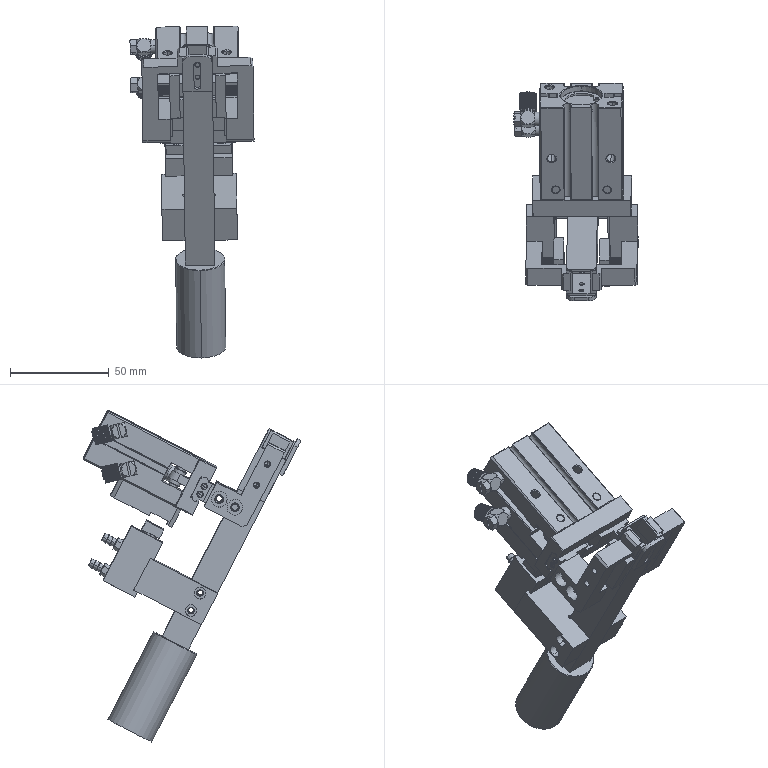Assembly | SolidWorks | mm | 18 component files | 21 solids | 1337 faces | box 62.86 x 110.43 x 168.21 mm | volume 158382 mm3 | plane 692 | cylinder 460 | cone 157 | spline 12 | sphere 12 | torus 4 | commonest cylinder face diameters 8.5 x72 2.5 x49 6 x38 3 x22 4.134 x20 5 x20 8 x20 4 x18
Bill of materials:
2018SOLIDWORKS1400000009 | 1 | 6061 Alloy | Rectangular block with a central rectangular slot that splits one end into two legs (a U/fork shape). It has a shallow step or lip along the top edges, small round relief grooves at the inner corners of the slot, and cross holes through the legs.
2018SOLIDWORKS1400000010 | 1 | 45 Steel | Long, narrow flat bar or channel that comes out of a short solid cylinder at one end. The far end splits into two thin prongs with small holes, and there is a pair of small holes partway along the bar.
2018SOLIDWORKS1400000011 | 1 | Black POM | Flat rectangular plate with two rounded corners on one end and one long obround slot through it.
2018SOLIDWORKS1400000012 | 1 | 45 Steel | L-shaped stepped bracket with an extra notched tab at the tip of one arm. Several through holes run through the plate-like face, some with counterbore-like rims.
2018SOLIDWORKS1400000013 | 1 | 45 Steel | L-shaped stepped bracket with a notched tab at one arm end. It has two larger counterbored-looking holes at the corner end and two smaller holes along the long arm.
2018SOLIDWORKS1400000014 | 2 | White High Temperature Silicone | Plain rectangular block or thick plate with a shallow narrow rectangular step or groove near one edge.
2018SOLIDWORKS1400000015 | 2 | 45 Steel | Plain rectangular block or thick plate with no visible holes or other features.
2018SOLIDWORKS1400000016 | 1 | 6061 Alloy | Rectangular plate with chamfered corners. It has two plain through holes, two counterbored holes, and a stepped notch along one edge.
PurchasedPart;Three-axisCylinderTCM10x5S | 1 |  | Rectangular block with two parallel vertical slots that have semicircular ends. It also has a lateral groove, a row of holes and counterbores on one face, and side holes. A thin plate on a short neck stands off one end.
PurchasedPart_5mmSmallSpring | 2 |  | Helical coil of round wire with many evenly spaced turns. A solid cylinder sits inside part of its length.
PurchasedPart_MiniConnector03-_4 | 2 |  | Axially symmetric tubular fitting-like part. It has a hex flange, a short plain spigot on one side and a tapered, ringed (barb-like) stem on the other, with a through bore.
PurchasedPart_MS-5HLH-6StainlessSteelConnector | 2 |  | Compact body with a rounded or spherical central section. A hex section with a slot sits on one side and a stepped cylindrical nozzle with a bore on the opposite side. A large knurled or fluted cylindrical knob comes out at a right angle.
Y0365088900012 | 1 |  | Rectangular prismatic body with a wider transverse plate across one end. Two parallel rectangular jaw-like fingers stick out of that end. The overall shape looks like a two-finger parallel gripper unit.
Mates:
1. distance | 2018SOLIDWORKS1400000015-1 face at (82.559, -98.378, 177.003) dir (-0.9999, 0, -0.01383) | 2018SOLIDWORKS1400000012-1 face at (76.322, -113.007, 194.123) dir (0.9999, 0, 0.01383)
2. concentric | 2018SOLIDWORKS1400000012-1 face at (70.561, -98.378, 176.837) dir (0.9999, 0, 0.01383) r 3 | 2018SOLIDWORKS1400000015-1 face at (85.559, -98.378, 177.045) dir (-0.9999, 0, -0.01383) r 2.5
3. parallel | 2018SOLIDWORKS1400000012-1 face at (68.765, -96.483, 162.032) dir (0.00635, -0.8884, -0.459) | 2018SOLIDWORKS1400000015-1 face at (82.755, -99.533, 162.901) dir (0.00635, -0.8884, -0.459)
4. coincident | 2018SOLIDWORKS1400000012-1 face at (75.885, -87.155, 153.442) dir (0.9999, 0, 0.01383) | Y0365088900012-1 face at (75.284, -13.933, 196.896) dir (-0.9999, 0, -0.01383)
5. concentric | 2018SOLIDWORKS1400000012-1 face at (68.79, -84.741, 160.22) dir (-0.9999, 0, -0.01383) r 2.25 | Y0365088900012-1 face at (79.794, -84.741, 160.372) dir (0.9999, 0, 0.01383) r 1.621
6. concentric | 2018SOLIDWORKS1400000012-1 face at (68.733, -76.745, 164.351) dir (-0.9999, 0, -0.01383) r 2.25 | Y0365088900012-1 face at (79.737, -76.745, 164.503) dir (0.9999, 0, 0.01383) r 1.621
7. coincident | Y0365088900012-1 face at (117.579, -13.933, 197.481) dir (0.9999, 0, 0.01383) | 2018SOLIDWORKS1400000013-1 face at (118.072, -82.786, 161.912) dir (-0.9999, 0, -0.01383)
8. concentric | Y0365088900012-1 face at (114.024, -76.745, 164.977) dir (0.9999, 0, 0.01383) r 1.621 | 2018SOLIDWORKS1400000013-1 face at (125.028, -76.745, 165.129) dir (0.9999, 0, 0.01383) r 2.25
9. concentric | Y0365088900012-1 face at (114.081, -84.741, 160.846) dir (0.9999, 0, 0.01383) r 1.621 | 2018SOLIDWORKS1400000013-1 face at (125.085, -84.741, 160.999) dir (0.9999, 0, 0.01383) r 2.25
10. distance | 2018SOLIDWORKS1400000015-2 face at (110.859, -98.645, 177.257) dir (0.9999, 0, 0.01383) | 2018SOLIDWORKS1400000013-1 face at (116.618, -113.007, 194.681) dir (-0.9999, 0, -0.01383)
11. concentric | 2018SOLIDWORKS1400000013-1 face at (122.857, -98.645, 177.423) dir (-0.9999, 0, -0.01383) r 3 | 2018SOLIDWORKS1400000015-2 face at (107.859, -98.645, 177.216) dir (0.9999, 0, 0.01383) r 2.5
12. parallel | 2018SOLIDWORKS1400000015-1 face at (82.755, -99.533, 162.901) dir (0.00635, -0.8884, -0.459) | 2018SOLIDWORKS1400000015-2 face at (111.054, -99.8, 163.155) dir (0.00635, -0.8884, -0.459)
13. concentric | 2018SOLIDWORKS1400000013-1 face at (122.857, -98.645, 177.423) dir (-0.9999, 0, -0.01383) r 3 | PurchasedPart_5mmSmallSpring-2 face at (117.858, -98.645, 177.354) dir (0.9999, 0, 0.01383) r 1.5
14. coincident | 2018SOLIDWORKS1400000013-1 face at (122.857, -98.645, 177.423) dir (-0.9999, 0, -0.01383) | PurchasedPart_5mmSmallSpring-2 face at (122.857, -98.645, 177.423) dir (0.9999, 0, 0.01383)
15. concentric | 2018SOLIDWORKS1400000012-1 face at (70.561, -98.378, 176.837) dir (0.9999, 0, 0.01383) r 3 | PurchasedPart_5mmSmallSpring-1 face at (75.56, -98.378, 176.907) dir (-0.9999, 0, -0.01383) r 1.5
16. coincident | 2018SOLIDWORKS1400000012-1 face at (70.561, -98.378, 176.837) dir (0.9999, 0, 0.01383) | PurchasedPart_5mmSmallSpring-1 face at (70.561, -98.378, 176.837) dir (-0.9999, 0, -0.01383)
17. coincident | 2018SOLIDWORKS1400000012-1 face at (88.833, -112.548, 193.408) dir (0.01229, 0.459, -0.8883) | 2018SOLIDWORKS1400000014-1 face at (91.802, -108.284, 195.653) dir (-0.01229, -0.459, 0.8883)
18. width | 2018SOLIDWORKS1400000014-1 face at (88.834, -114.314, 193.34) dir (0.00635, -0.8884, -0.459) | 2018SOLIDWORKS1400000014-1 face at (88.753, -102.942, 199.215) dir (-0.00635, 0.8884, 0.459) | 2018SOLIDWORKS1400000012-1 face at (68.262, -104.478, 198.419) dir (-0.00635, 0.8884, 0.459) | 2018SOLIDWORKS1400000012-1 face at (68.765, -96.483, 162.032) dir (0.00635, -0.8884, -0.459)
19. coincident | 2018SOLIDWORKS1400000012-1 face at (89.274, -82.786, 161.513) dir (0.9999, 0, 0.01383) | 2018SOLIDWORKS1400000014-1 face at (88.852, -106.448, 192.058) dir (-0.9999, 0, -0.01383)
20. coincident | 2018SOLIDWORKS1400000013-1 face at (104.573, -82.786, 161.725) dir (-0.9999, 0, -0.01383) | 2018SOLIDWORKS1400000014-2 face at (104.15, -106.448, 192.269) dir (0.9999, 0, 0.01383)
21. coincident | 2018SOLIDWORKS1400000013-1 face at (104.071, -104.019, 198.026) dir (0.01229, 0.459, -0.8883) | 2018SOLIDWORKS1400000014-2 face at (101.101, -108.284, 195.781) dir (-0.01229, -0.459, 0.8883)
22. width | 2018SOLIDWORKS1400000014-2 face at (104.051, -102.942, 199.426) dir (-0.00635, 0.8884, 0.459) | 2018SOLIDWORKS1400000014-2 face at (104.133, -114.314, 193.552) dir (0.00635, -0.8884, -0.459) | 2018SOLIDWORKS1400000013-1 face at (125.232, -90.057, 150.374) dir (0.00635, -0.8884, -0.459) | 2018SOLIDWORKS1400000013-1 face at (124.556, -104.478, 199.198) dir (-0.00635, 0.8884, 0.459)
23. distance | PurchasedPart;Three-axisCylinderTCM10x5S-1 face at (97.066, -44.276, 151.351) dir (-0.01229, -0.459, 0.8883) | 2018SOLIDWORKS1400000016-1 face at (96.944, -38.131, 160.153) dir (0.01229, 0.459, -0.8883)
24. coincident | PurchasedPart;Three-axisCylinderTCM10x5S-1 face at (113.657, -46.423, 144.842) dir (0.00635, -0.8884, -0.459) | 2018SOLIDWORKS1400000016-1 face at (76.038, -51.013, 153.207) dir (-0.00635, 0.8884, 0.459)
25. width | PurchasedPart;Three-axisCylinderTCM10x5S-1 face at (80.66, -46.423, 144.386) dir (-0.9999, 0, -0.01383) | PurchasedPart;Three-axisCylinderTCM10x5S-1 face at (113.594, -37.539, 149.432) dir (0.9999, 0, 0.01383) | 2018SOLIDWORKS1400000016-1 face at (117.955, -57.351, 159.518) dir (0.9999, 0, 0.01383) | 2018SOLIDWORKS1400000016-1 face at (75.959, -57.351, 158.937) dir (-0.9999, 0, -0.01383)
26. coincident | Y0365088900012-1 face at (87.752, -7.599, 184.807) dir (0.01229, 0.459, -0.8883) | 2018SOLIDWORKS1400000016-1 face at (96.846, -41.803, 167.259) dir (-0.01229, -0.459, 0.8883)
27. width | Y0365088900012-1 face at (75.594, -7.923, 185.267) dir (-0.9999, 0, -0.01383) | Y0365088900012-1 face at (117.456, -12.958, 195.592) dir (0.9999, 0, 0.01383) | 2018SOLIDWORKS1400000016-1 face at (117.955, -57.351, 159.518) dir (0.9999, 0, 0.01383) | 2018SOLIDWORKS1400000016-1 face at (75.959, -57.351, 158.937) dir (-0.9999, 0, -0.01383)
28. concentric | Y0365088900012-1 face at (81.723, -35.758, 176.046) dir (-0.01229, -0.459, 0.8883) r 2.067 | 2018SOLIDWORKS1400000016-1 face at (81.91, -28.773, 162.529) dir (0.01229, 0.459, -0.8883) r 2.75
29. concentric | Y0365088900012-1 face at (111.72, -35.758, 176.461) dir (-0.01229, -0.459, 0.8883) r 2.067 | 2018SOLIDWORKS1400000016-1 face at (111.907, -28.773, 162.944) dir (0.01229, 0.459, -0.8883) r 2.75
30. coincident | 2018SOLIDWORKS1400000010-1 face at (88.967, -116.186, 194.569) dir (0.00635, -0.8884, -0.459) | 2018SOLIDWORKS1400000011-1 face at (96.491, -111.826, 186.233) dir (-0.00635, 0.8884, 0.459)
31. parallel | 2018SOLIDWORKS1400000010-1 face at (88.872, -102.86, 201.454) dir (-0.9999, 0, -0.01383) | 2018SOLIDWORKS1400000011-1 face at (88.868, -116.416, 195.012) dir (-0.9999, 0, -0.01383)
32. width | Y0365088900012-1 face at (75.407, -14.908, 198.785) dir (-0.9999, 0, -0.01383) | Y0365088900012-1 face at (117.269, -19.943, 209.11) dir (0.9999, 0, 0.01383) | 2018SOLIDWORKS1400000010-1 face at (103.966, -116.186, 194.777) dir (0.9999, 0, 0.01383) | 2018SOLIDWORKS1400000010-1 face at (88.872, -102.86, 201.454) dir (-0.9999, 0, -0.01383)
33. distance | 2018SOLIDWORKS1400000011-1 face at (88.868, -116.416, 195.012) dir (-0.01229, -0.459, 0.8883) | 2018SOLIDWORKS1400000010-1 face at (89.017, -119.94, 190.942) dir (-0.01229, -0.459, 0.8883)
34. distance | 2018SOLIDWORKS1400000009-1 face at (97.641, -50.659, 109.788) dir (0.01229, 0.459, -0.8883) | PurchasedPart;Three-axisCylinderTCM10x5S-1 face at (92.375, -20.896, 121.716) dir (0.01229, 0.459, -0.8883)
35. coincident | PurchasedPart;Three-axisCylinderTCM10x5S-1 face at (91.069, -33.956, 114.95) dir (0.00635, -0.8884, -0.459) | 2018SOLIDWORKS1400000009-1 face at (97.421, -39.464, 125.7) dir (-0.00635, 0.8884, 0.459)
36. width | 2018SOLIDWORKS1400000009-1 face at (116.295, -41.818, 134.876) dir (0.9999, 0, 0.01383) | 2018SOLIDWORKS1400000009-1 face at (78.299, -41.818, 134.35) dir (-0.9999, 0, -0.01383) | PurchasedPart;Three-axisCylinderTCM10x5S-1 face at (80.57, -33.956, 114.804) dir (-0.9999, 0, -0.01383) | PurchasedPart;Three-axisCylinderTCM10x5S-1 face at (114.452, -17.964, 123.536) dir (0.9999, 0, 0.01383)
37. coincident | 2018SOLIDWORKS1400000010-1 face at (103.87, -102.86, 201.661) dir (-0.00635, 0.8884, 0.459) | 2018SOLIDWORKS1400000009-1 face at (105.167, -54.435, 107.941) dir (0.00635, -0.8884, -0.459)
38. distance | 2018SOLIDWORKS1400000009-1 face at (97.641, -50.659, 109.788) dir (0.01229, 0.459, -0.8883) | 2018SOLIDWORKS1400000010-1 face at (97.894, -54.442, 91.514) dir (-0.01229, -0.459, 0.8883)
39. concentric | PurchasedPart;Three-axisCylinderTCM10x5S-1 face at (97.392, -20.259, 127.743) dir (0.00635, -0.8884, -0.459) r 1.23 | PurchasedPart_MiniConnector03-_4-1 face at (97.408, -22.481, 126.595) dir (-0.00635, 0.8884, 0.459) r 1.5
40. coincident | PurchasedPart;Three-axisCylinderTCM10x5S-1 face at (93.854, -17.964, 123.251) dir (-0.00635, 0.8884, 0.459) | PurchasedPart_MiniConnector03-_4-1 face at (97.392, -20.259, 127.743) dir (0.00635, -0.8884, -0.459)
41. concentric | PurchasedPart;Three-axisCylinderTCM10x5S-1 face at (97.214, -26.915, 140.624) dir (0.00635, -0.8884, -0.459) r 1.23 | PurchasedPart_MiniConnector03-_4-2 face at (97.23, -29.136, 139.476) dir (-0.00635, 0.8884, 0.459) r 1.5
42. coincident | PurchasedPart;Three-axisCylinderTCM10x5S-1 face at (93.854, -17.964, 123.251) dir (-0.00635, 0.8884, 0.459) | PurchasedPart_MiniConnector03-_4-2 face at (97.214, -26.915, 140.624) dir (0.00635, -0.8884, -0.459)
43. concentric | Y0365088900012-1 face at (78.119, -25.993, 199.146) dir (-0.9999, 0, -0.01383) r 2.067 | PurchasedPart_MS-5HLH-6StainlessSteelConnector-1 face at (76.658, -25.993, 199.126) dir (-0.9999, 0, -0.01383) r 2.5
44. coincident | Y0365088900012-1 face at (75.407, -14.908, 198.785) dir (-0.9999, 0, -0.01383) | PurchasedPart_MS-5HLH-6StainlessSteelConnector-1 face at (75.394, -28.917, 199.783) dir (0.9999, 0, 0.01383)
45. coincident | Y0365088900012-1 face at (75.594, -7.923, 185.267) dir (-0.9999, 0, -0.01383) | PurchasedPart_MS-5HLH-6StainlessSteelConnector-2 face at (75.662, -33.848, 180.353) dir (0.9999, 0, 0.01383)
46. concentric | Y0365088900012-1 face at (78.388, -30.924, 179.717) dir (-0.9999, 0, -0.01383) r 2.067 | PurchasedPart_MS-5HLH-6StainlessSteelConnector-2 face at (74.422, -30.924, 179.662) dir (-0.9999, 0, -0.01383) r 3.5